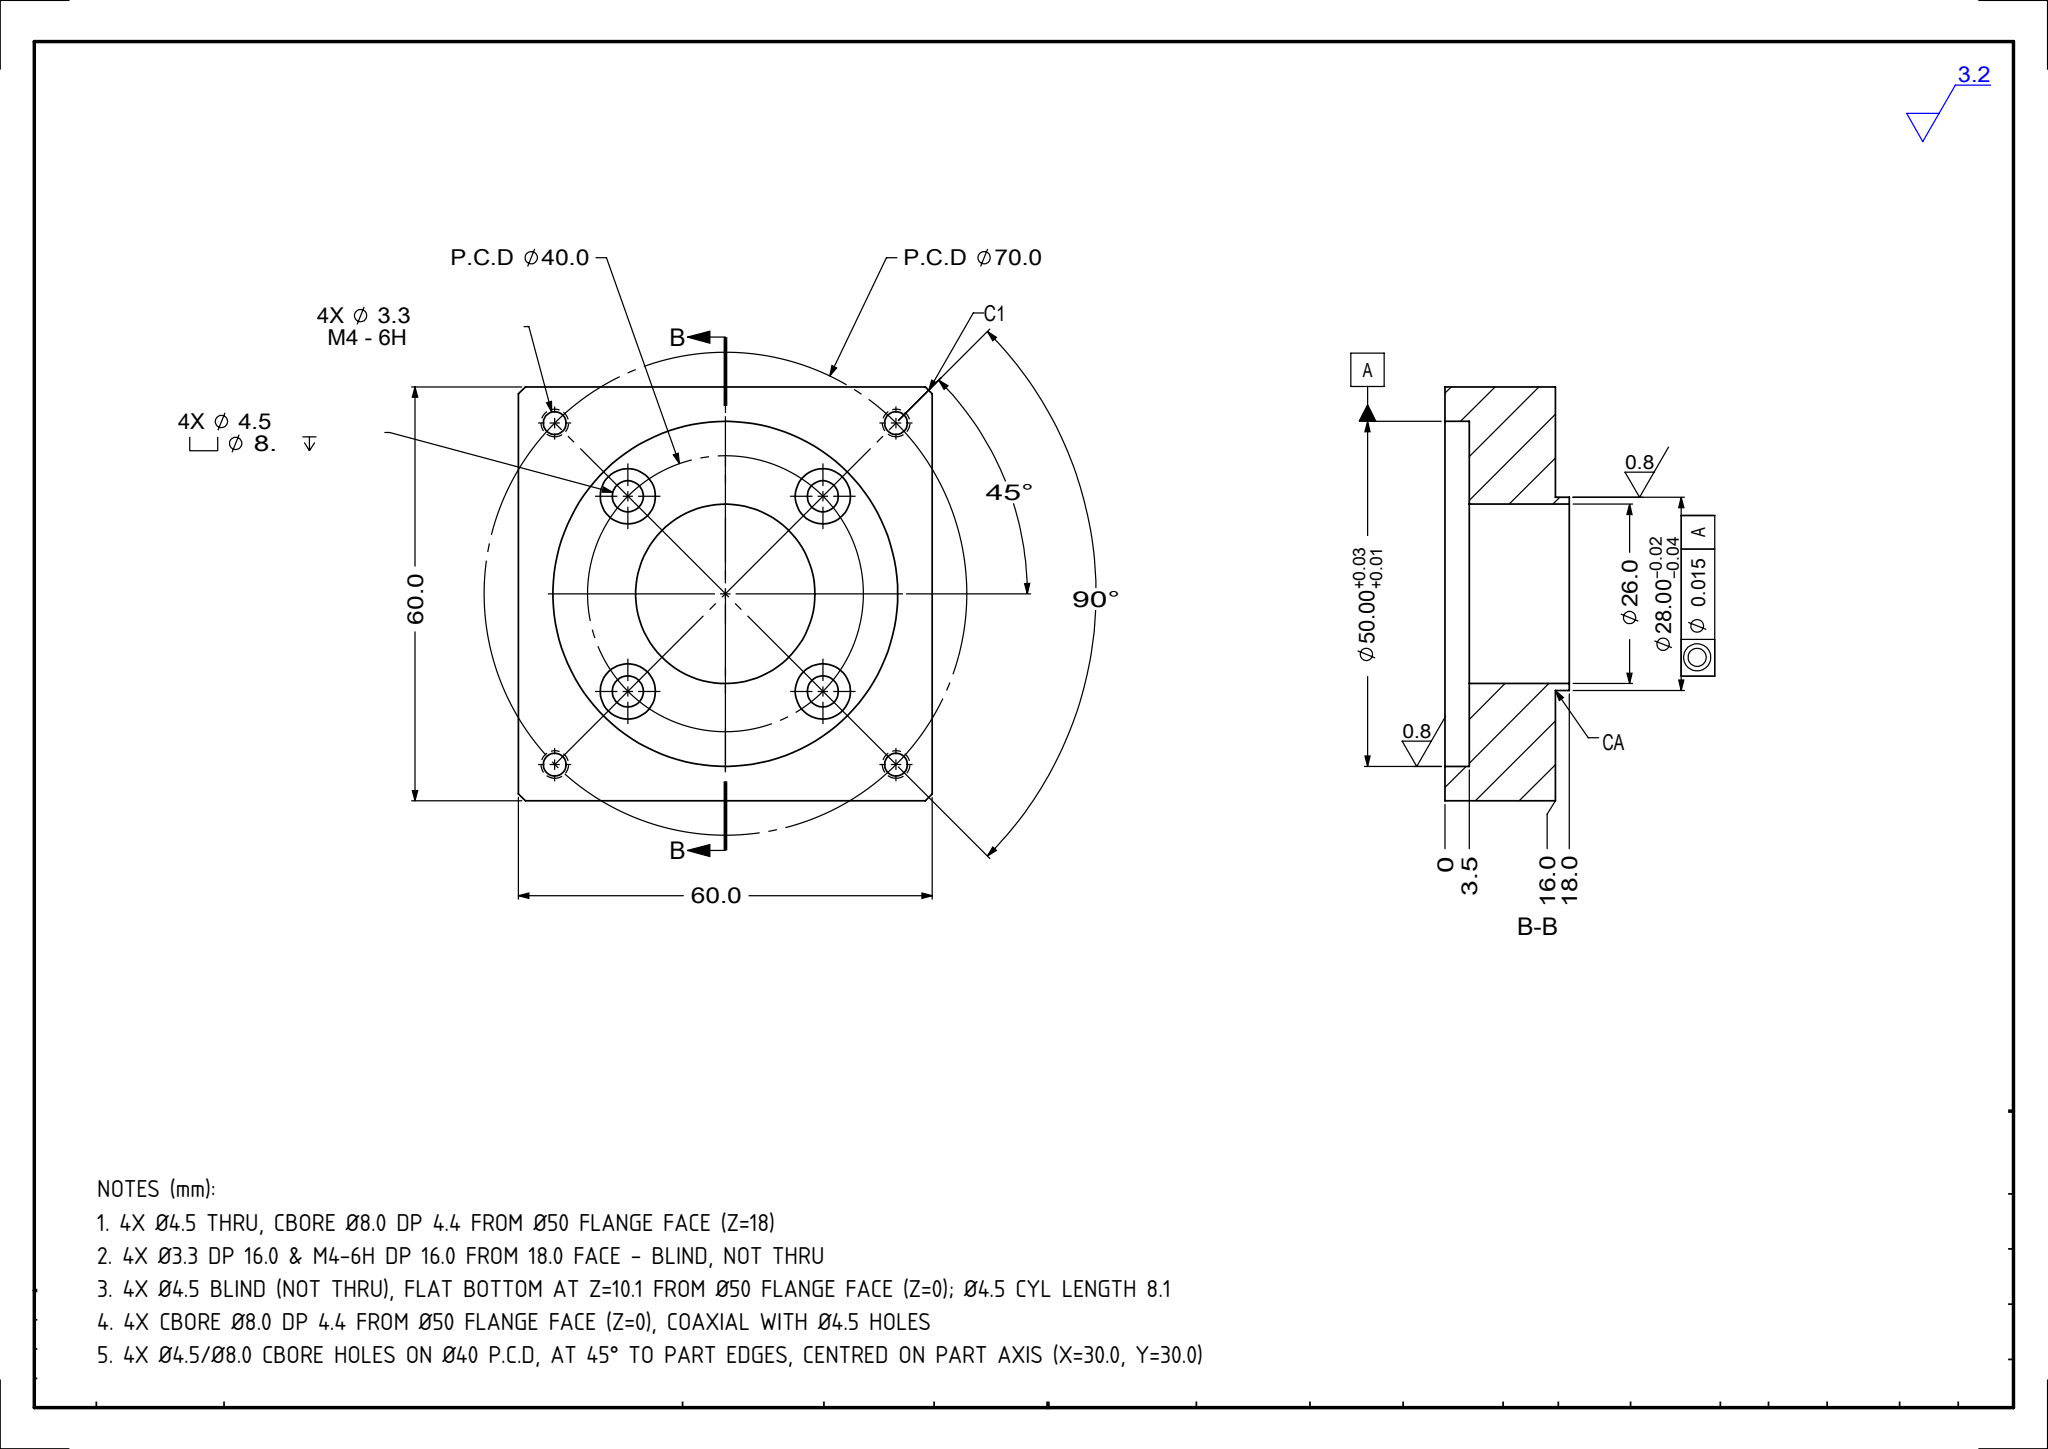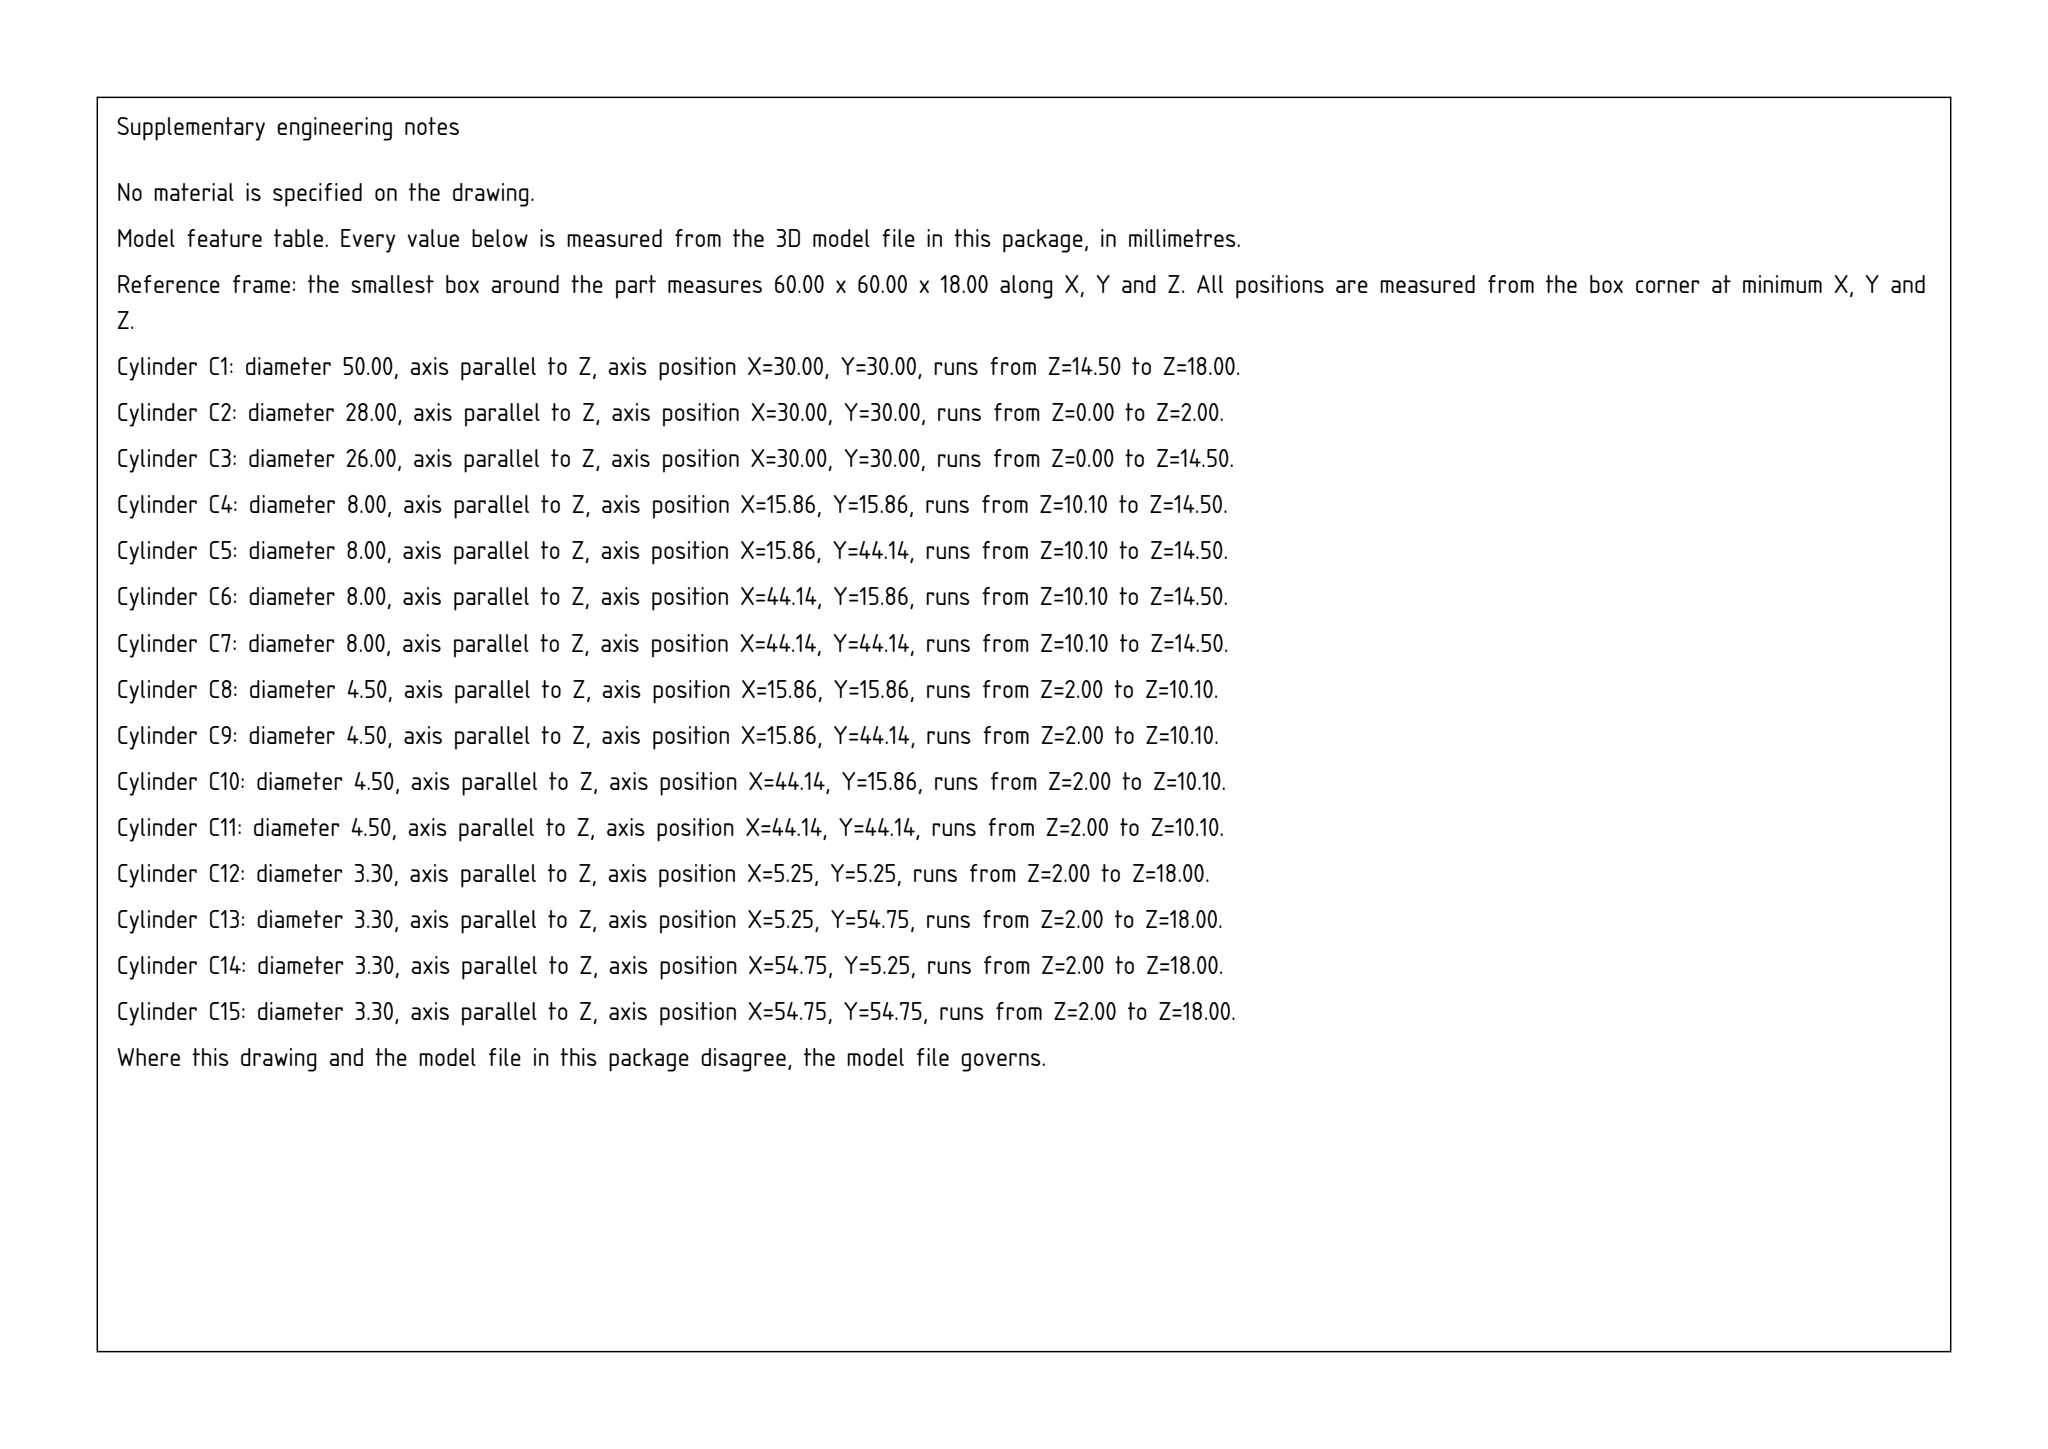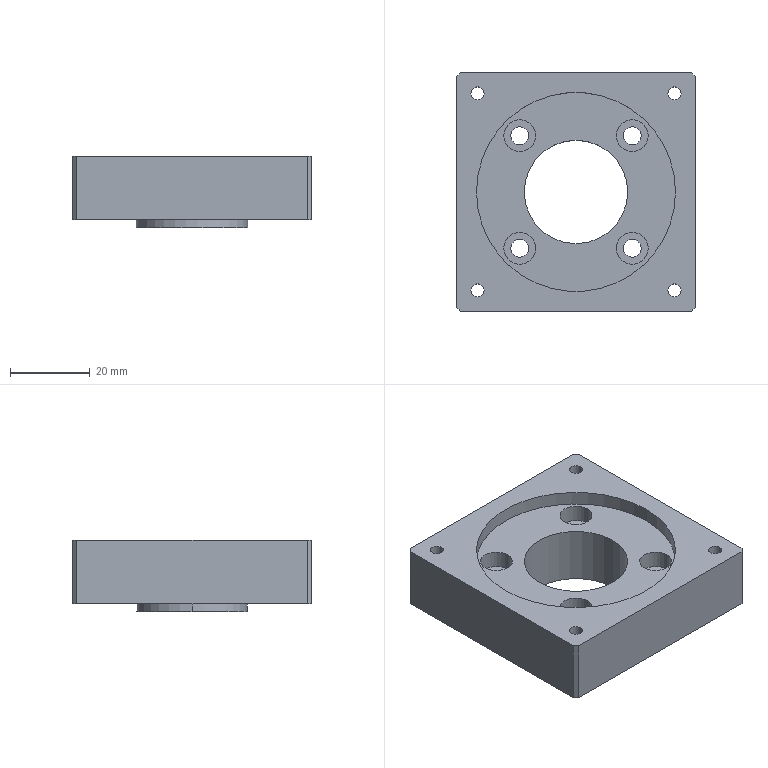Part | SolidWorks | mm | 1 solid | 46 faces | box 60 x 60 x 18 mm | volume 42281 mm3 | cylinder 30 | plane 16 | commonest cylinder face diameters 3.3 x8 8 x8 4.5 x8 50 x2 28 x2 26 x2
Drawing notes:
4X Ø4.5 THRU, CBORE Ø8.0 DP 4.4 FROM Ø50 FLANGE FACE (Z=18) | from the solid: cyl Ø8.0 L=4.4 at (15.86/44.14,15.86/44.14), z-plane 10.1 to 14.5; Ø4.5 L=8.1 thru; flange face Ø50 at z=14.5-18.0
4X Ø3.3 DP 16.0 & M4-6H DP 16.0 FROM 18.0 FACE - BLIND, NOT THRU | from the solid: cylinders [3.3,"z",(5.25,5.25),(5.25,54.75),(54.75,5.25),(54.75,54.75), length 16.0] in 18.0 thick part (z planes 0.0 and 18.0); PCD70 corner holes
4X Ø4.5 BLIND (NOT THRU), FLAT BOTTOM AT Z=10.1 FROM Ø50 FLANGE FACE (Z=0); Ø4.5 CYL LENGTH 8.1 | from the solid: cylinders [4.5,z,(15.86/44.14,15.86/44.14),len 8.1] x4 with axis_plane z=10.1 (4 flat bottoms), part bbox z=18.0
4X CBORE Ø8.0 DP 4.4 FROM Ø50 FLANGE FACE (Z=0), COAXIAL WITH Ø4.5 HOLES | from the solid: cylinders [8.0,z,(15.86/44.14,15.86/44.14),len 4.4] x4; Ø50 flange z=0 to 3.5
4X Ø4.5/Ø8.0 CBORE HOLES ON Ø40 P.C.D, AT 45° TO PART EDGES, CENTRED ON PART AXIS (X=30.0, Y=30.0) | from the solid: cylinder centres (15.86,15.86),(15.86,44.14),(44.14,15.86),(44.14,44.14) vs bbox 60x60 centre (30,30) → radius 20.0
build123d program:
from build123d import *

# Parameters (mm, degrees)
SKETCH1_W                                       = 60
SKETCH1_H                                       = 60
BOSS_EXTRUDE1_DEPTH                             = 9
SKETCH2_W                                       = 60
SKETCH2_H                                       = 60
SKETCH2_R                                       = 14
CUT_EXTRUDE1_DEPTH                              = 2
SKETCH3_R                                       = 13
CUT_EXTRUDE2_DEPTH                              = 47.087
SKETCH4_R                                       = 25
CUT_EXTRUDE3_DEPTH                              = 3.5
CHAMFER1_SIZE                                   = 1
M4_HEX_SOCKET_HEAD_CAP_SCREW_CBORE1_D           = 4.5
M4_HEX_SOCKET_HEAD_CAP_SCREW_CBORE1_CBORE_D     = 8
M4_HEX_SOCKET_HEAD_CAP_SCREW_CBORE1_CBORE_DEPTH = 4.4
M4_TAPPED_HOLE2_D                               = 3.3


with BuildPart() as part:
    # Sketch1 → Boss-Extrude1 (new, symmetric)
    with BuildSketch(Plane.XY):
        Rectangle(SKETCH1_W, SKETCH1_H)
    extrude(amount=BOSS_EXTRUDE1_DEPTH, both=True)

    # Sketch2 → Cut-Extrude1 (cut)
    with BuildSketch(Plane(origin=(0, 0, -9), x_dir=(-1, 0, 0), z_dir=(0, 0, -1))):
        Rectangle(SKETCH2_W, SKETCH2_H)
        Circle(SKETCH2_R, mode=Mode.SUBTRACT)
    extrude(amount=-CUT_EXTRUDE1_DEPTH, mode=Mode.SUBTRACT)

    # Sketch3 → Cut-Extrude2 (cut, through all)
    with BuildSketch(Plane(origin=(0, 0, -9), x_dir=(-1, 0, 0), z_dir=(0, 0, -1))):
        Circle(SKETCH3_R)
    extrude(amount=-CUT_EXTRUDE2_DEPTH, mode=Mode.SUBTRACT)

    # Sketch4 → Cut-Extrude3 (cut)
    with BuildSketch(Plane.XY.offset(9)):
        Circle(SKETCH4_R)
    extrude(amount=-CUT_EXTRUDE3_DEPTH, mode=Mode.SUBTRACT)

    # Chamfer1
    chamfer1_edges = [part.edges().sort_by_distance(p)[0] for p in [
        (30, -30, 1),
        (-30, -30, 1),
        (-30, 30, 1),
        (30, 30, 1),
    ]]
    chamfer(chamfer1_edges, length=CHAMFER1_SIZE)

    # M4 Hex Socket Head Cap Screw CBORE1 (through all)
    with Locations(Plane.XY.offset(5.5)):
        with Locations((14.142, -14.142), (14.142, 14.142), (-14.142, -14.142), (-14.142, 14.142)):
            CounterBoreHole(M4_HEX_SOCKET_HEAD_CAP_SCREW_CBORE1_D / 2, M4_HEX_SOCKET_HEAD_CAP_SCREW_CBORE1_CBORE_D / 2, M4_HEX_SOCKET_HEAD_CAP_SCREW_CBORE1_CBORE_DEPTH)

    # M4 Tapped Hole2 (through all)
    with Locations(Plane.XY.offset(9)):
        with Locations((-24.749, 24.749), (24.749, 24.749), (-24.749, -24.749), (24.749, -24.749)):
            Hole(M4_TAPPED_HOLE2_D / 2)


solid = part.part